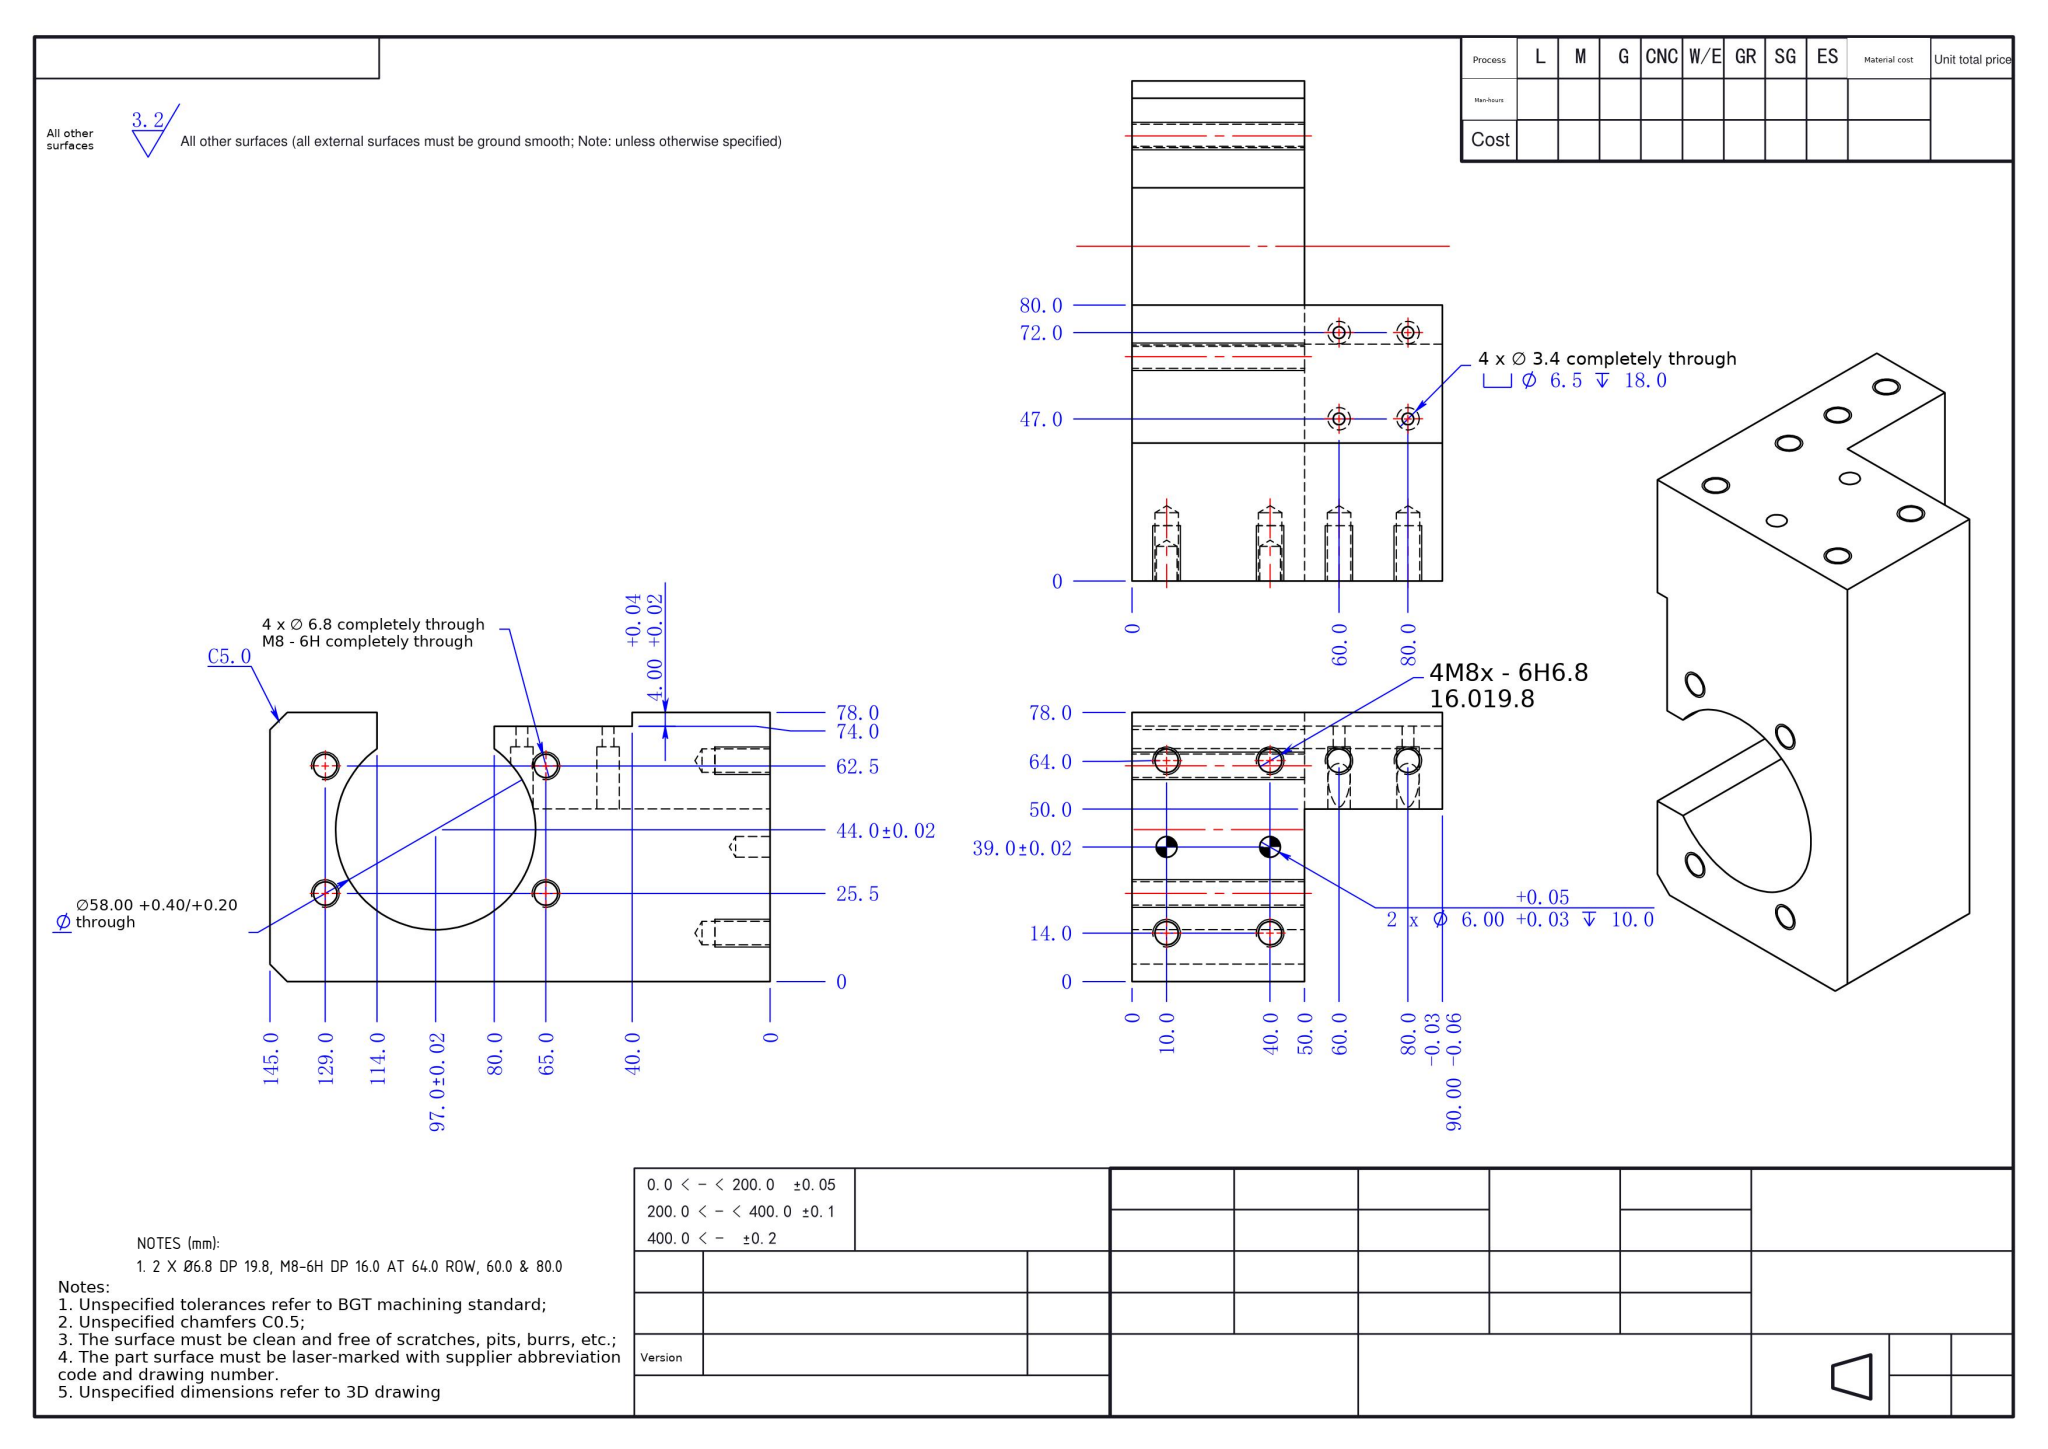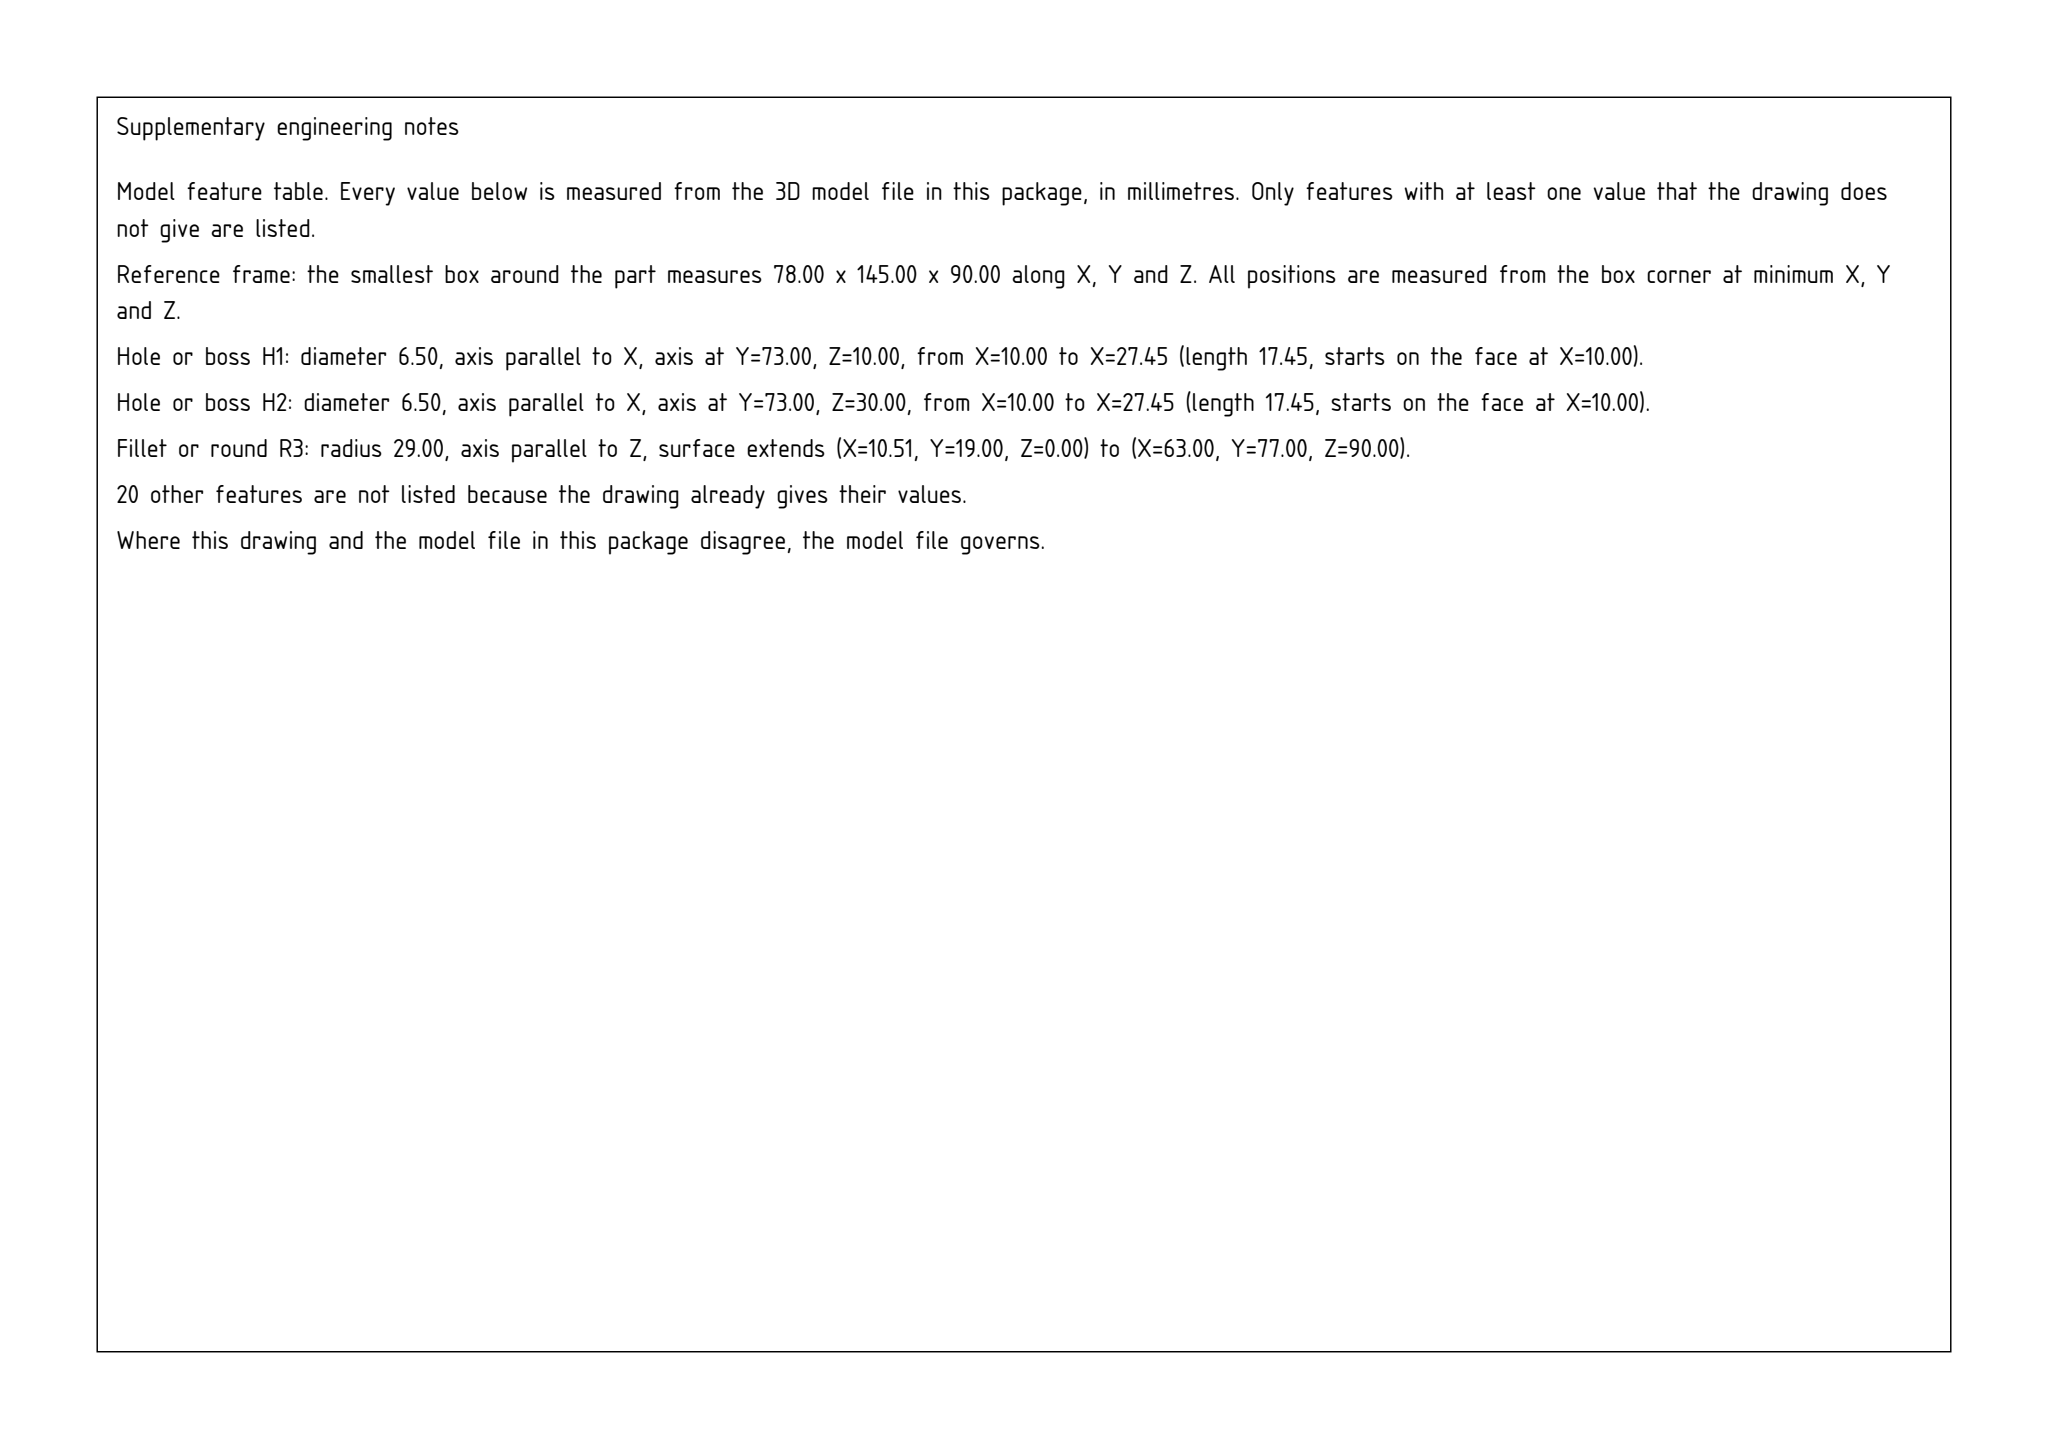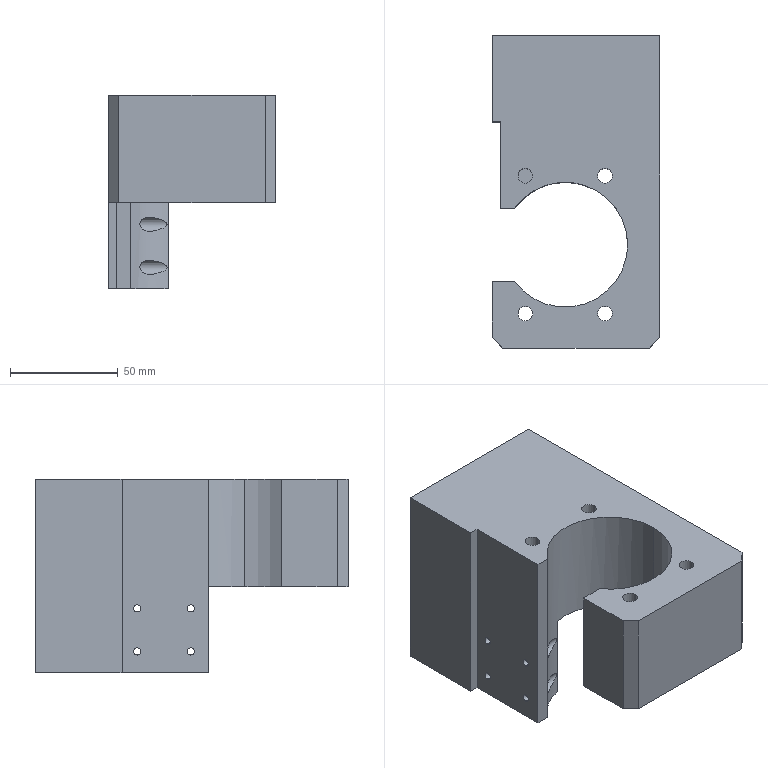Part | SolidWorks | mm | 1 solid | 78 faces | box 78 x 145 x 90 mm | volume 476418 mm3 | cylinder 42 | plane 20 | cone 16 | commonest cylinder face diameters 6.8 x20 6.5 x8 3.4 x8 6 x4 58 x2
Drawing notes:
2 X Ø6.8 DP 19.8, M8-6H DP 16.0 AT 64.0 ROW, 60.0 & 80.0 | from the solid: Ø6.8 Y-axis cyls at [x=14, z=10] and [x=14, z=30], L=19.75 w/ 118° point; mirrors the 4 called-out Ø6.8 Y holes at x=14/64, z=50/80 (drawing rows 64.0/14.0, pos 10.0/40.0)
build123d program:
from build123d import *

# Parameters (mm, degrees)
SKETCH1_W                                       = 68
SKETCH1_H                                       = 145
BOSS_EXTRUDE1_DEPTH                             = 50
SKETCH2_R                                       = 29
CUT_EXTRUDE1_DEPTH                              = 168.777
SKETCH3_W                                       = 50
SKETCH3_H                                       = 145
BOSS_EXTRUDE2_DEPTH                             = 10
SKETCH4_W                                       = 17.98
SKETCH4_H                                       = 34
CUT_EXTRUDE2_DEPTH                              = 173.073
M8_TAPPED_HOLE1_D                               = 6.8
M8_TAPPED_HOLE2_D                               = 6.8
M8_TAPPED_HOLE2_DEPTH                           = 19.75
M8_TAPPED_HOLE2_TIP                             = 2.043
SIZE_MM_DOWEL_HOLE1_D                           = 6
SIZE_MM_DOWEL_HOLE1_DEPTH                       = 10
SIZE_MM_DOWEL_HOLE1_TIP                         = 1.803
CHAMFER1_SIZE                                   = 5
SKETCH15_W                                      = 28
SKETCH15_H                                      = 80
BOSS_EXTRUDE3_DEPTH                             = 40
CUT_EXTRUDE3_DEPTH                              = 173.073
M3_HEX_SOCKET_HEAD_CAP_SCREW_CBORE1_D           = 3.4
M3_HEX_SOCKET_HEAD_CAP_SCREW_CBORE1_CBORE_D     = 6.5
M3_HEX_SOCKET_HEAD_CAP_SCREW_CBORE1_CBORE_DEPTH = 18
M8_TAPPED_HOLE3_D                               = 6.8
M8_TAPPED_HOLE3_DEPTH                           = 19.75
M8_TAPPED_HOLE3_TIP                             = 2.043
SKETCH22_W                                      = 4
SKETCH22_H                                      = 40
CUT_EXTRUDE5_DEPTH                              = 188.641


with BuildPart() as part:
    # Sketch1 → Boss-Extrude1 (new body)
    with BuildSketch(Plane.XY):
        with Locations((34, 72.5)):
            Rectangle(SKETCH1_W, SKETCH1_H)
    extrude(amount=BOSS_EXTRUDE1_DEPTH)

    # Sketch2 → Cut-Extrude1 (cut, through all)
    with BuildSketch(Plane.XY.offset(50)):
        with Locations((34, 48)):
            Circle(SKETCH2_R)
    extrude(amount=-CUT_EXTRUDE1_DEPTH, mode=Mode.SUBTRACT)

    # Sketch3 → Boss-Extrude2 (add)
    with BuildSketch(Plane(origin=(68, 0, 0), x_dir=(0, 0, -1), z_dir=(1, 0, 0))):
        with Locations((-25, 72.5)):
            Rectangle(SKETCH3_W, SKETCH3_H)
    extrude(amount=BOSS_EXTRUDE2_DEPTH)

    # Sketch4 → Cut-Extrude2 (cut, through all)
    with BuildSketch(Plane.XY.offset(50)):
        with Locations((8.99, 48)):
            Rectangle(SKETCH4_W, SKETCH4_H)
    extrude(amount=-CUT_EXTRUDE2_DEPTH, mode=Mode.SUBTRACT)

    # M8 Tapped Hole1 (through all)
    with Locations(Plane.XY.offset(50)):
        with Locations((15.5, 16), (52.5, 16), (52.5, 80), (15.5, 80)):
            Hole(M8_TAPPED_HOLE1_D / 2)

    # M8 Tapped Hole2
    with Locations(Plane(origin=(0, 145, 0), x_dir=(1, 0, 0), z_dir=(0, 1, 0))):
        with Locations((64, -40), (64, -10), (14, -40), (14, -10)):
            Hole(M8_TAPPED_HOLE2_D / 2, depth=M8_TAPPED_HOLE2_DEPTH)
            with Locations((0, 0, -(M8_TAPPED_HOLE2_DEPTH + M8_TAPPED_HOLE2_TIP / 2))):  # 118° drill point
                Cone(0, M8_TAPPED_HOLE2_D / 2, M8_TAPPED_HOLE2_TIP, mode=Mode.SUBTRACT)

    # Size mm Dowel Hole1
    with Locations(Plane(origin=(0, 145, 0), x_dir=(1, 0, 0), z_dir=(0, 1, 0))):
        with Locations((39, -40), (39, -10)):
            Hole(SIZE_MM_DOWEL_HOLE1_D / 2, depth=SIZE_MM_DOWEL_HOLE1_DEPTH)
            with Locations((0, 0, -(SIZE_MM_DOWEL_HOLE1_DEPTH + SIZE_MM_DOWEL_HOLE1_TIP / 2))):  # 118° drill point
                Cone(0, SIZE_MM_DOWEL_HOLE1_D / 2, SIZE_MM_DOWEL_HOLE1_TIP, mode=Mode.SUBTRACT)

    # Chamfer1
    chamfer1_edges = [part.edges().sort_by_distance(p)[0] for p in [
        (78, 0, 25),
        (0, 0, 25),
    ]]
    chamfer(chamfer1_edges, length=CHAMFER1_SIZE)

    # Sketch15 → Boss-Extrude3 (add)
    with BuildSketch(Plane(origin=(0, 0, 0), x_dir=(-1, 0, 0), z_dir=(0, 0, -1))):
        with Locations((-14, 105)):
            Rectangle(SKETCH15_W, SKETCH15_H)
    extrude(amount=BOSS_EXTRUDE3_DEPTH)

    # Sketch16 → Cut-Extrude3 (cut, through all)
    with BuildSketch(Plane.XY):
        with BuildLine():
            Line((28, 65), (28, 76.373))
            ThreePointArc((28, 76.373), (18.194, 72.314), (10.505, 65))
            Line((10.505, 65), (28, 65))
        make_face()
    extrude(amount=-CUT_EXTRUDE3_DEPTH, mode=Mode.SUBTRACT)

    # M3 Hex Socket Head Cap Screw CBORE1 (through all)
    with Locations(Plane(origin=(28, 0, 0), x_dir=(0, 0, -1), z_dir=(1, 0, 0))):
        with Locations((30, 98), (30, 73), (10, 98), (10, 73)):
            CounterBoreHole(M3_HEX_SOCKET_HEAD_CAP_SCREW_CBORE1_D / 2, M3_HEX_SOCKET_HEAD_CAP_SCREW_CBORE1_CBORE_D / 2, M3_HEX_SOCKET_HEAD_CAP_SCREW_CBORE1_CBORE_DEPTH)

    # M8 Tapped Hole3
    with Locations(Plane(origin=(0, 145, 0), x_dir=(1, 0, 0), z_dir=(0, 1, 0))):
        with Locations((14, 10), (14, 30)):
            Hole(M8_TAPPED_HOLE3_D / 2, depth=M8_TAPPED_HOLE3_DEPTH)
            with Locations((0, 0, -(M8_TAPPED_HOLE3_DEPTH + M8_TAPPED_HOLE3_TIP / 2))):  # 118° drill point
                Cone(0, M8_TAPPED_HOLE3_D / 2, M8_TAPPED_HOLE3_TIP, mode=Mode.SUBTRACT)

    # Sketch22 → Cut-Extrude5 (cut, through all)
    with BuildSketch(Plane(origin=(0, 0, -40), x_dir=(-1, 0, 0), z_dir=(0, 0, -1))):
        with Locations((-2, 85)):
            Rectangle(SKETCH22_W, SKETCH22_H)
    extrude(amount=-CUT_EXTRUDE5_DEPTH, mode=Mode.SUBTRACT)


solid = part.part